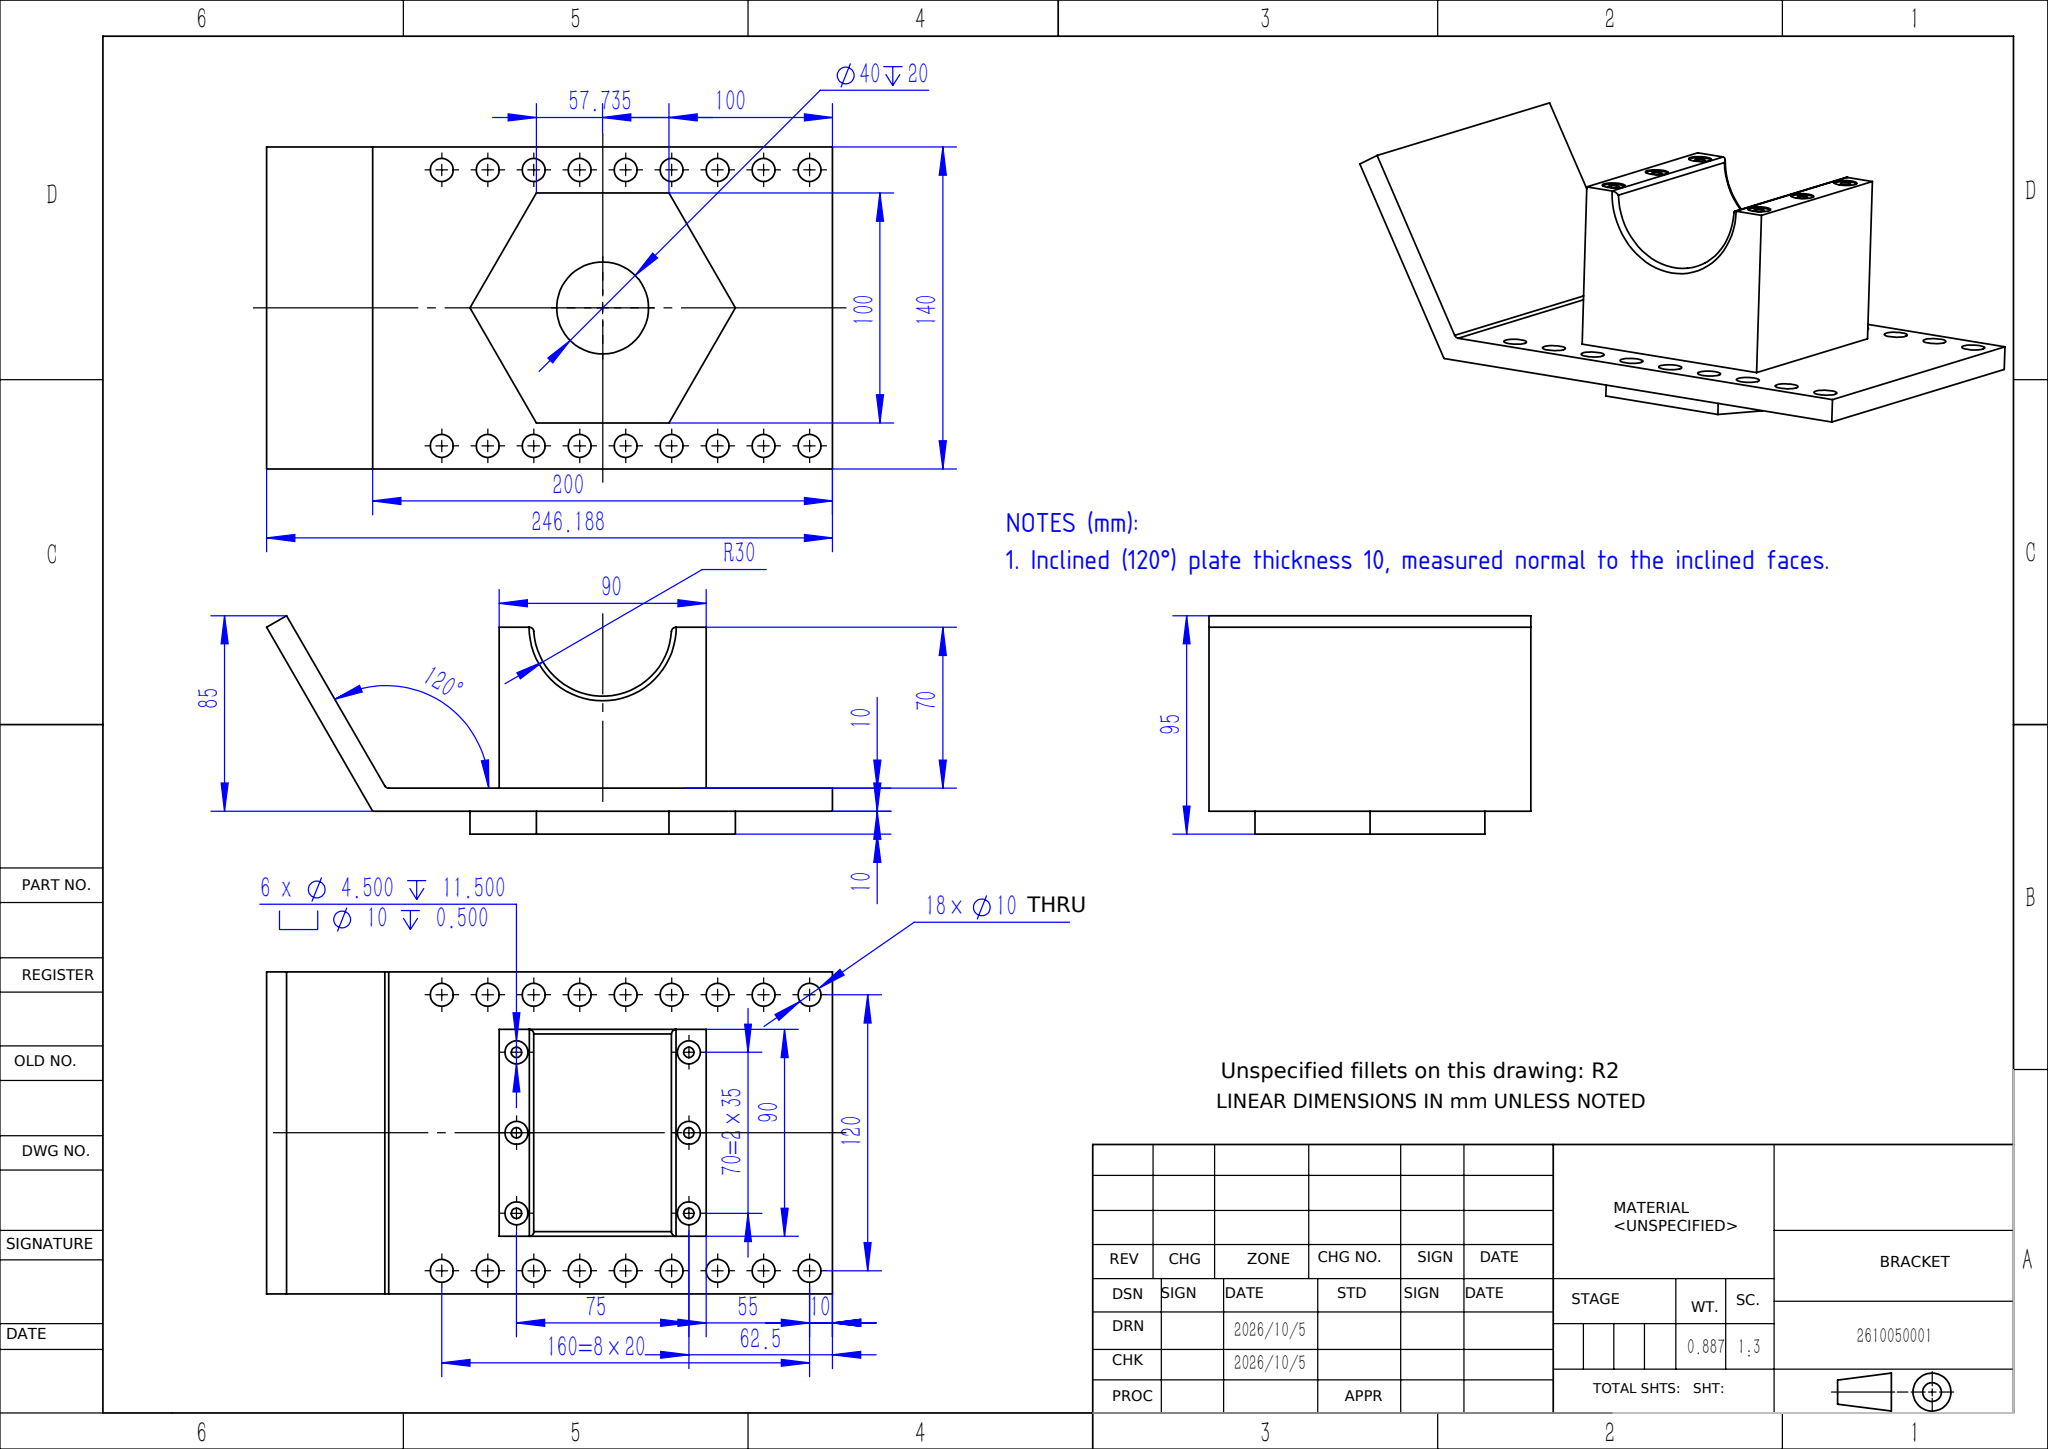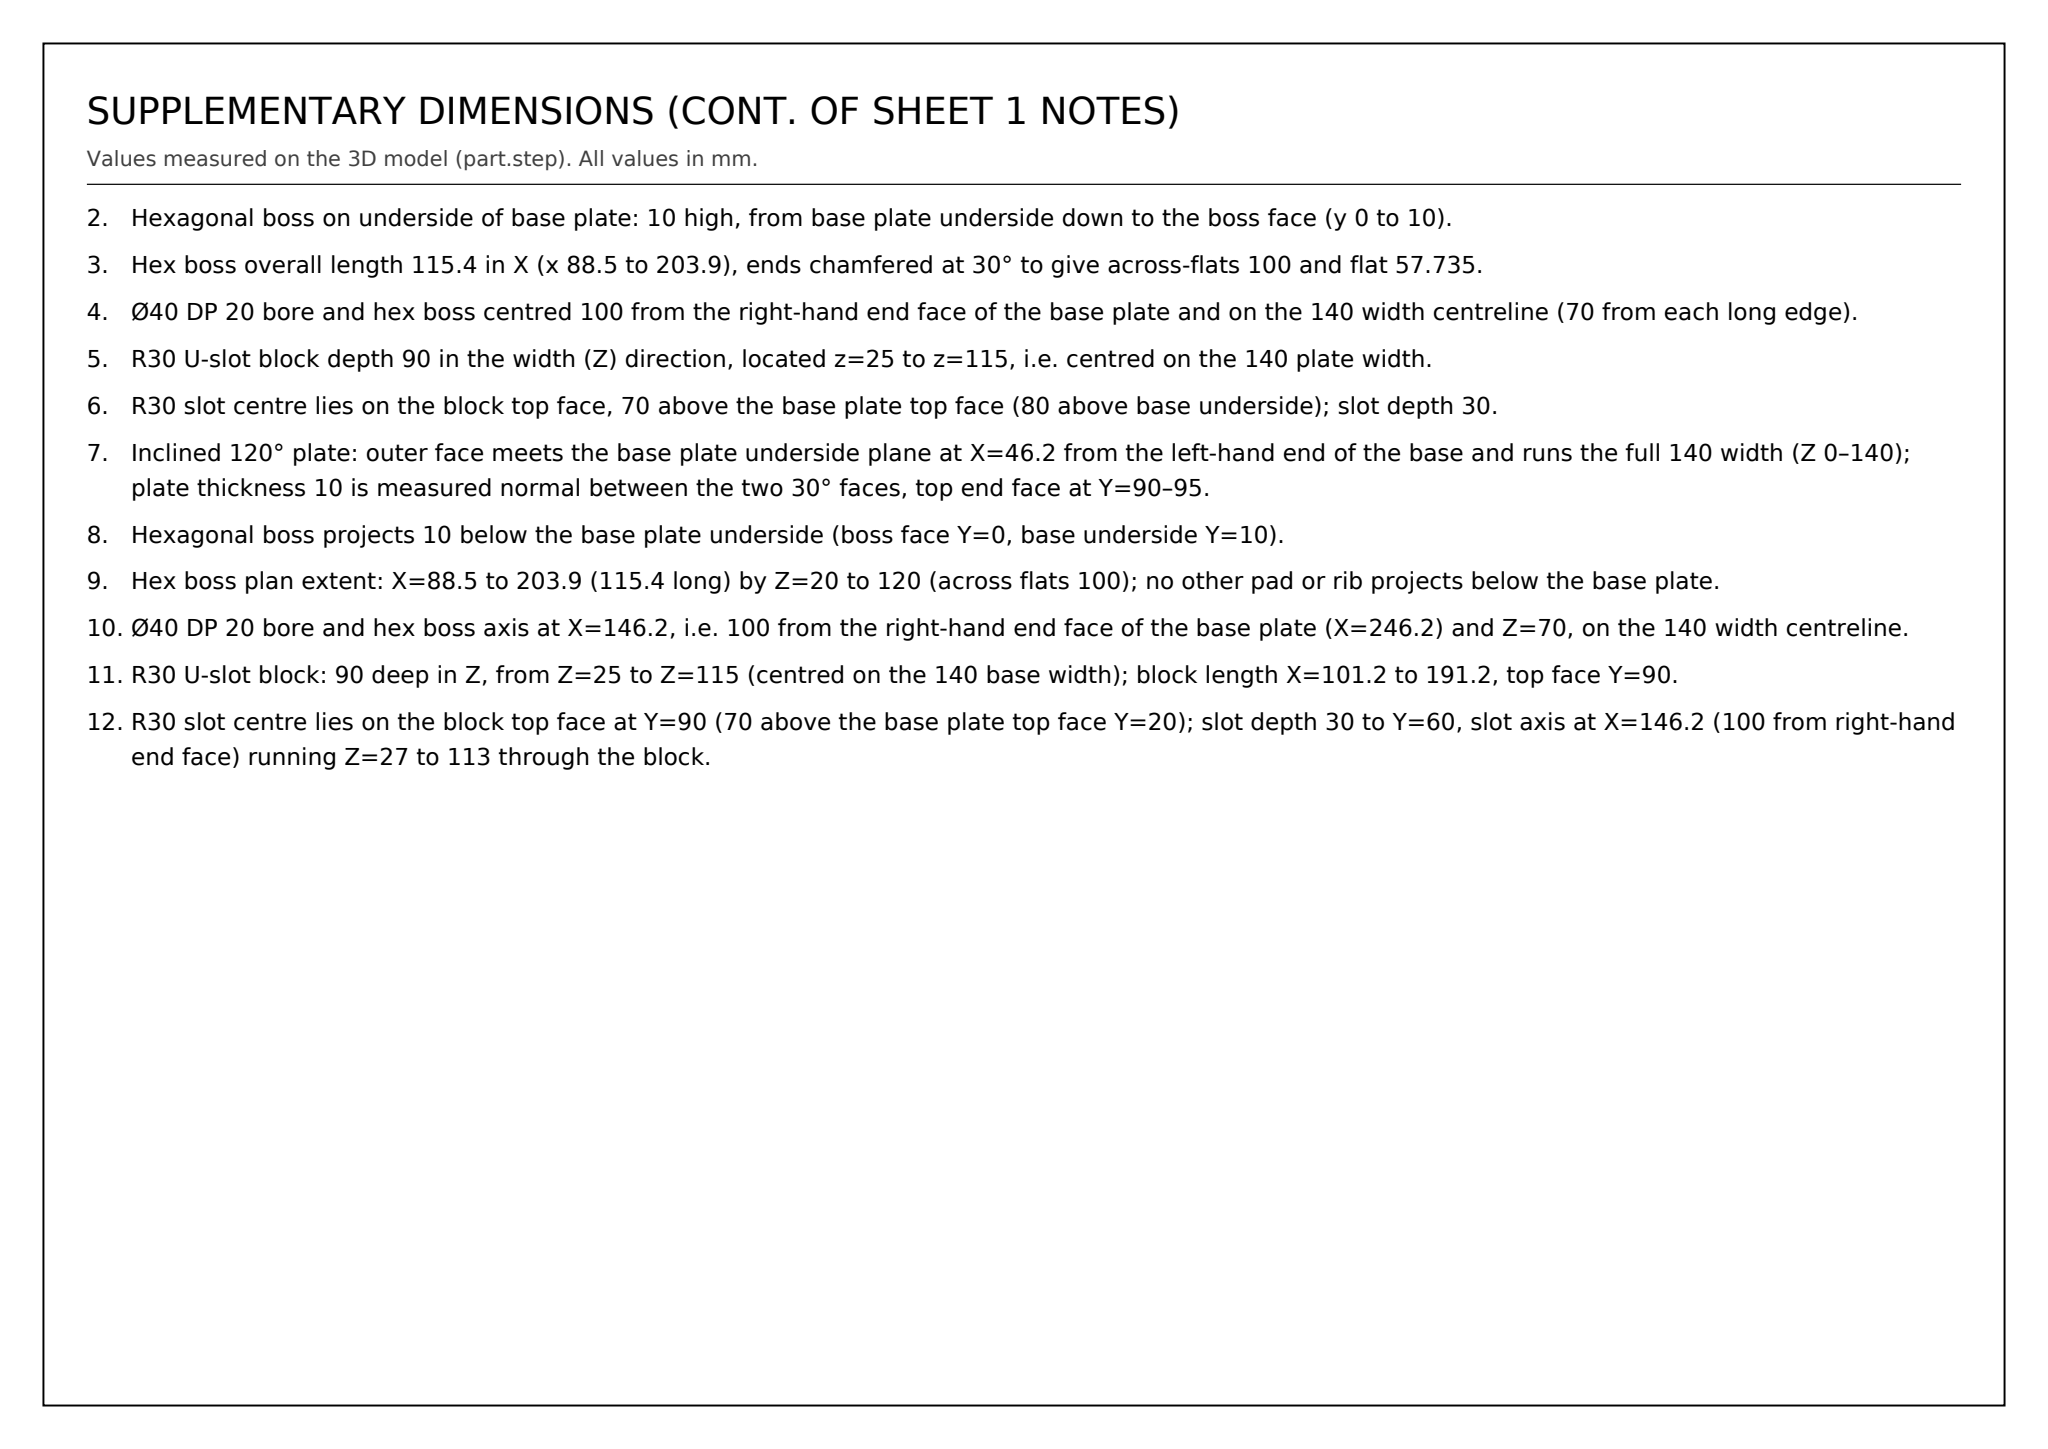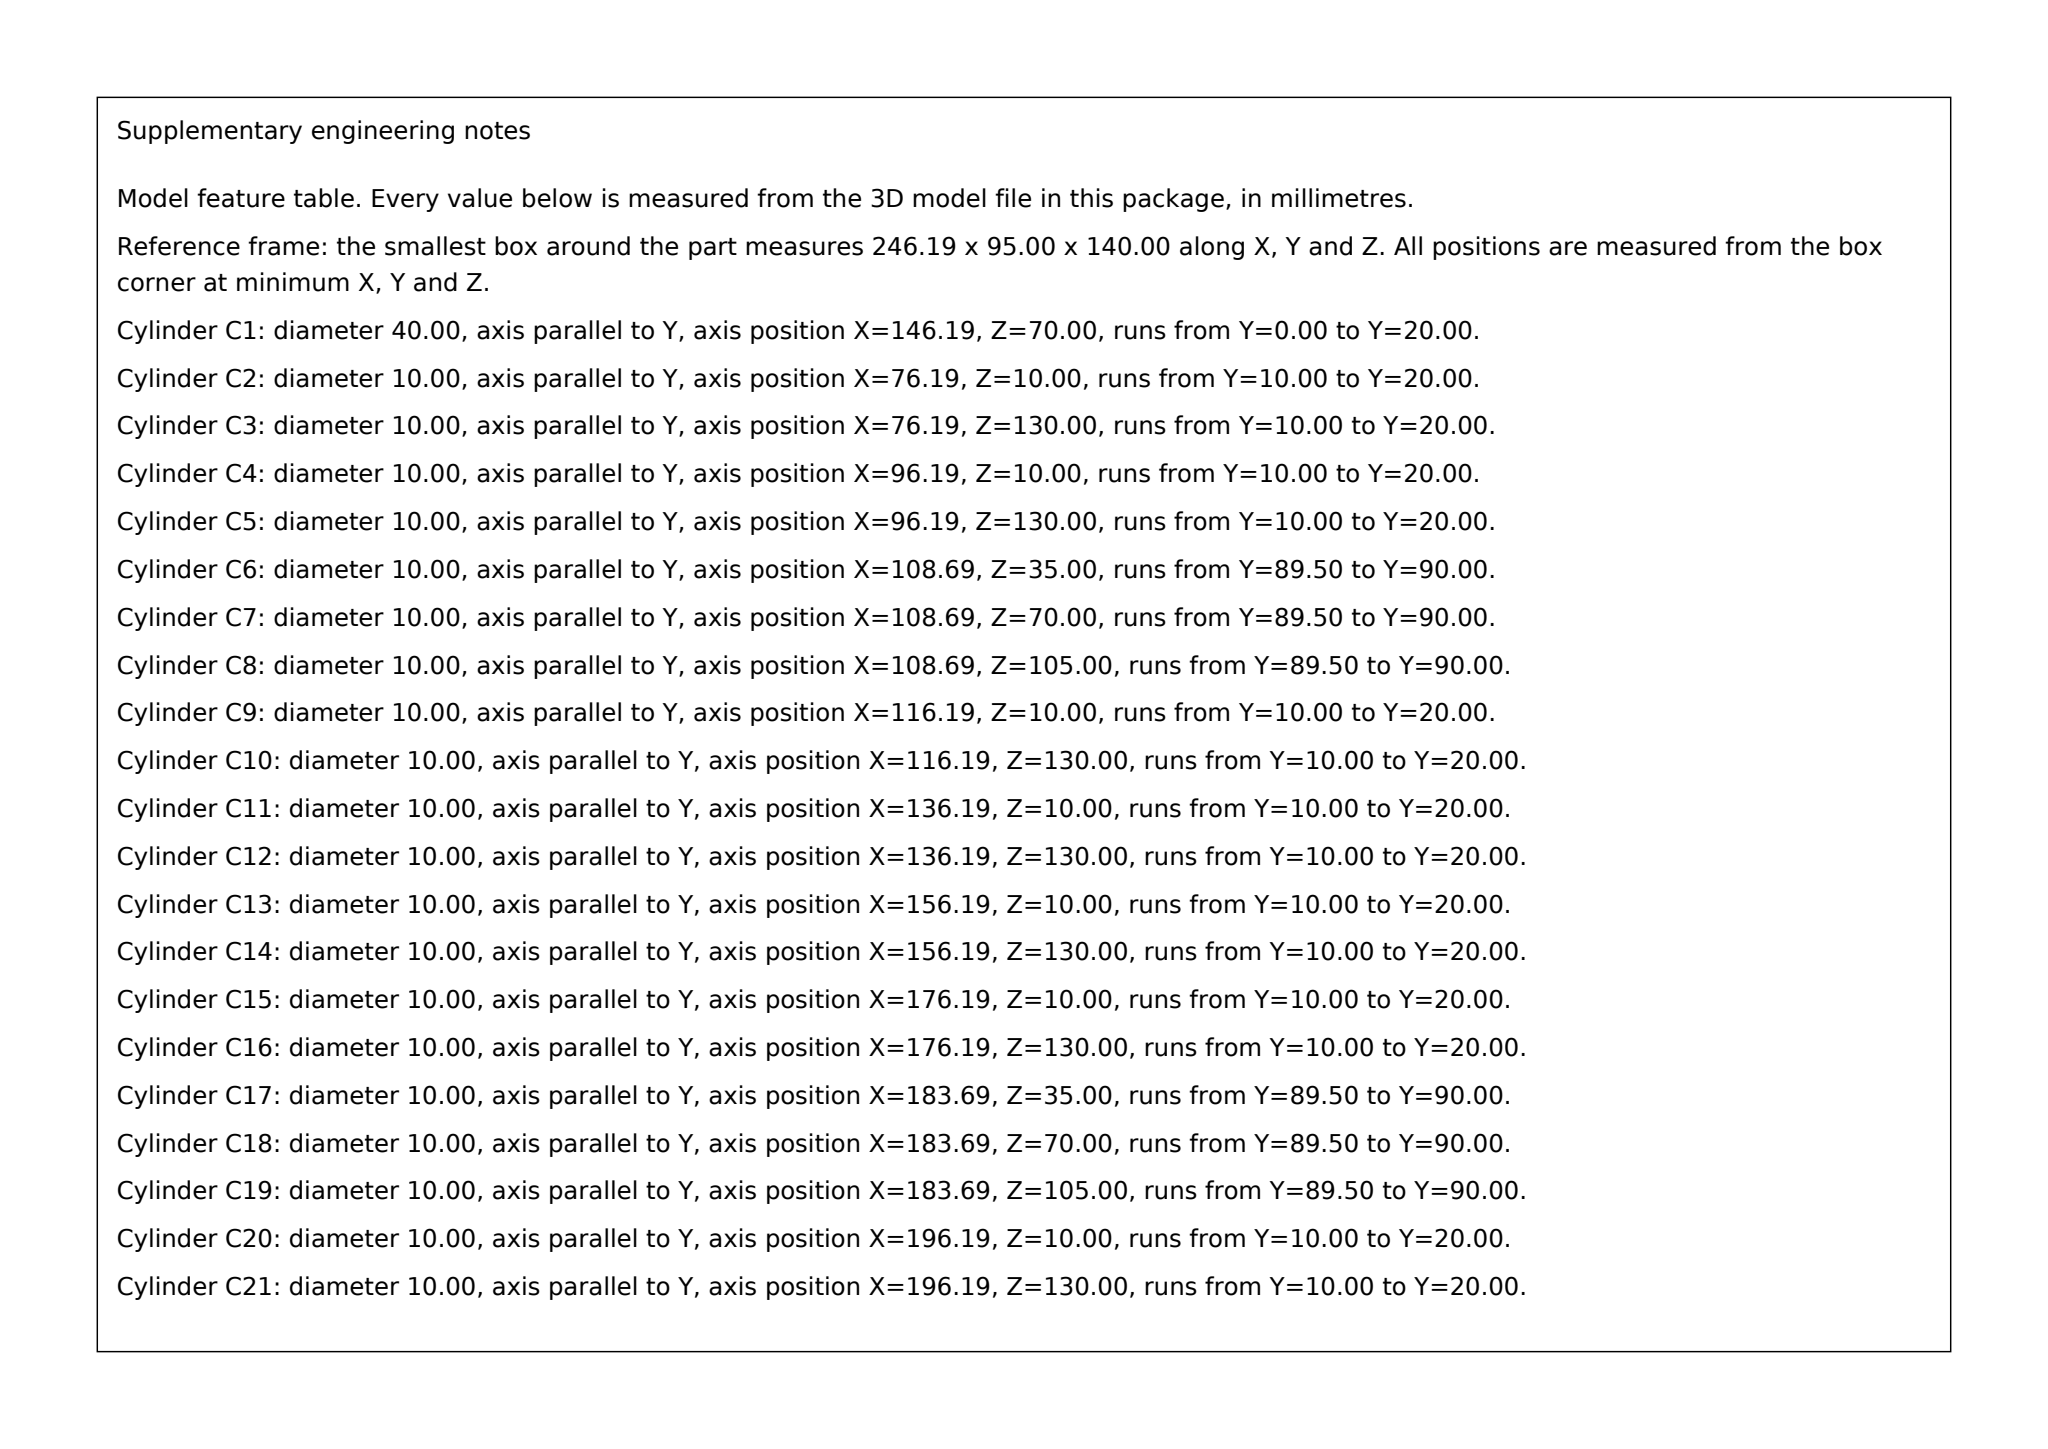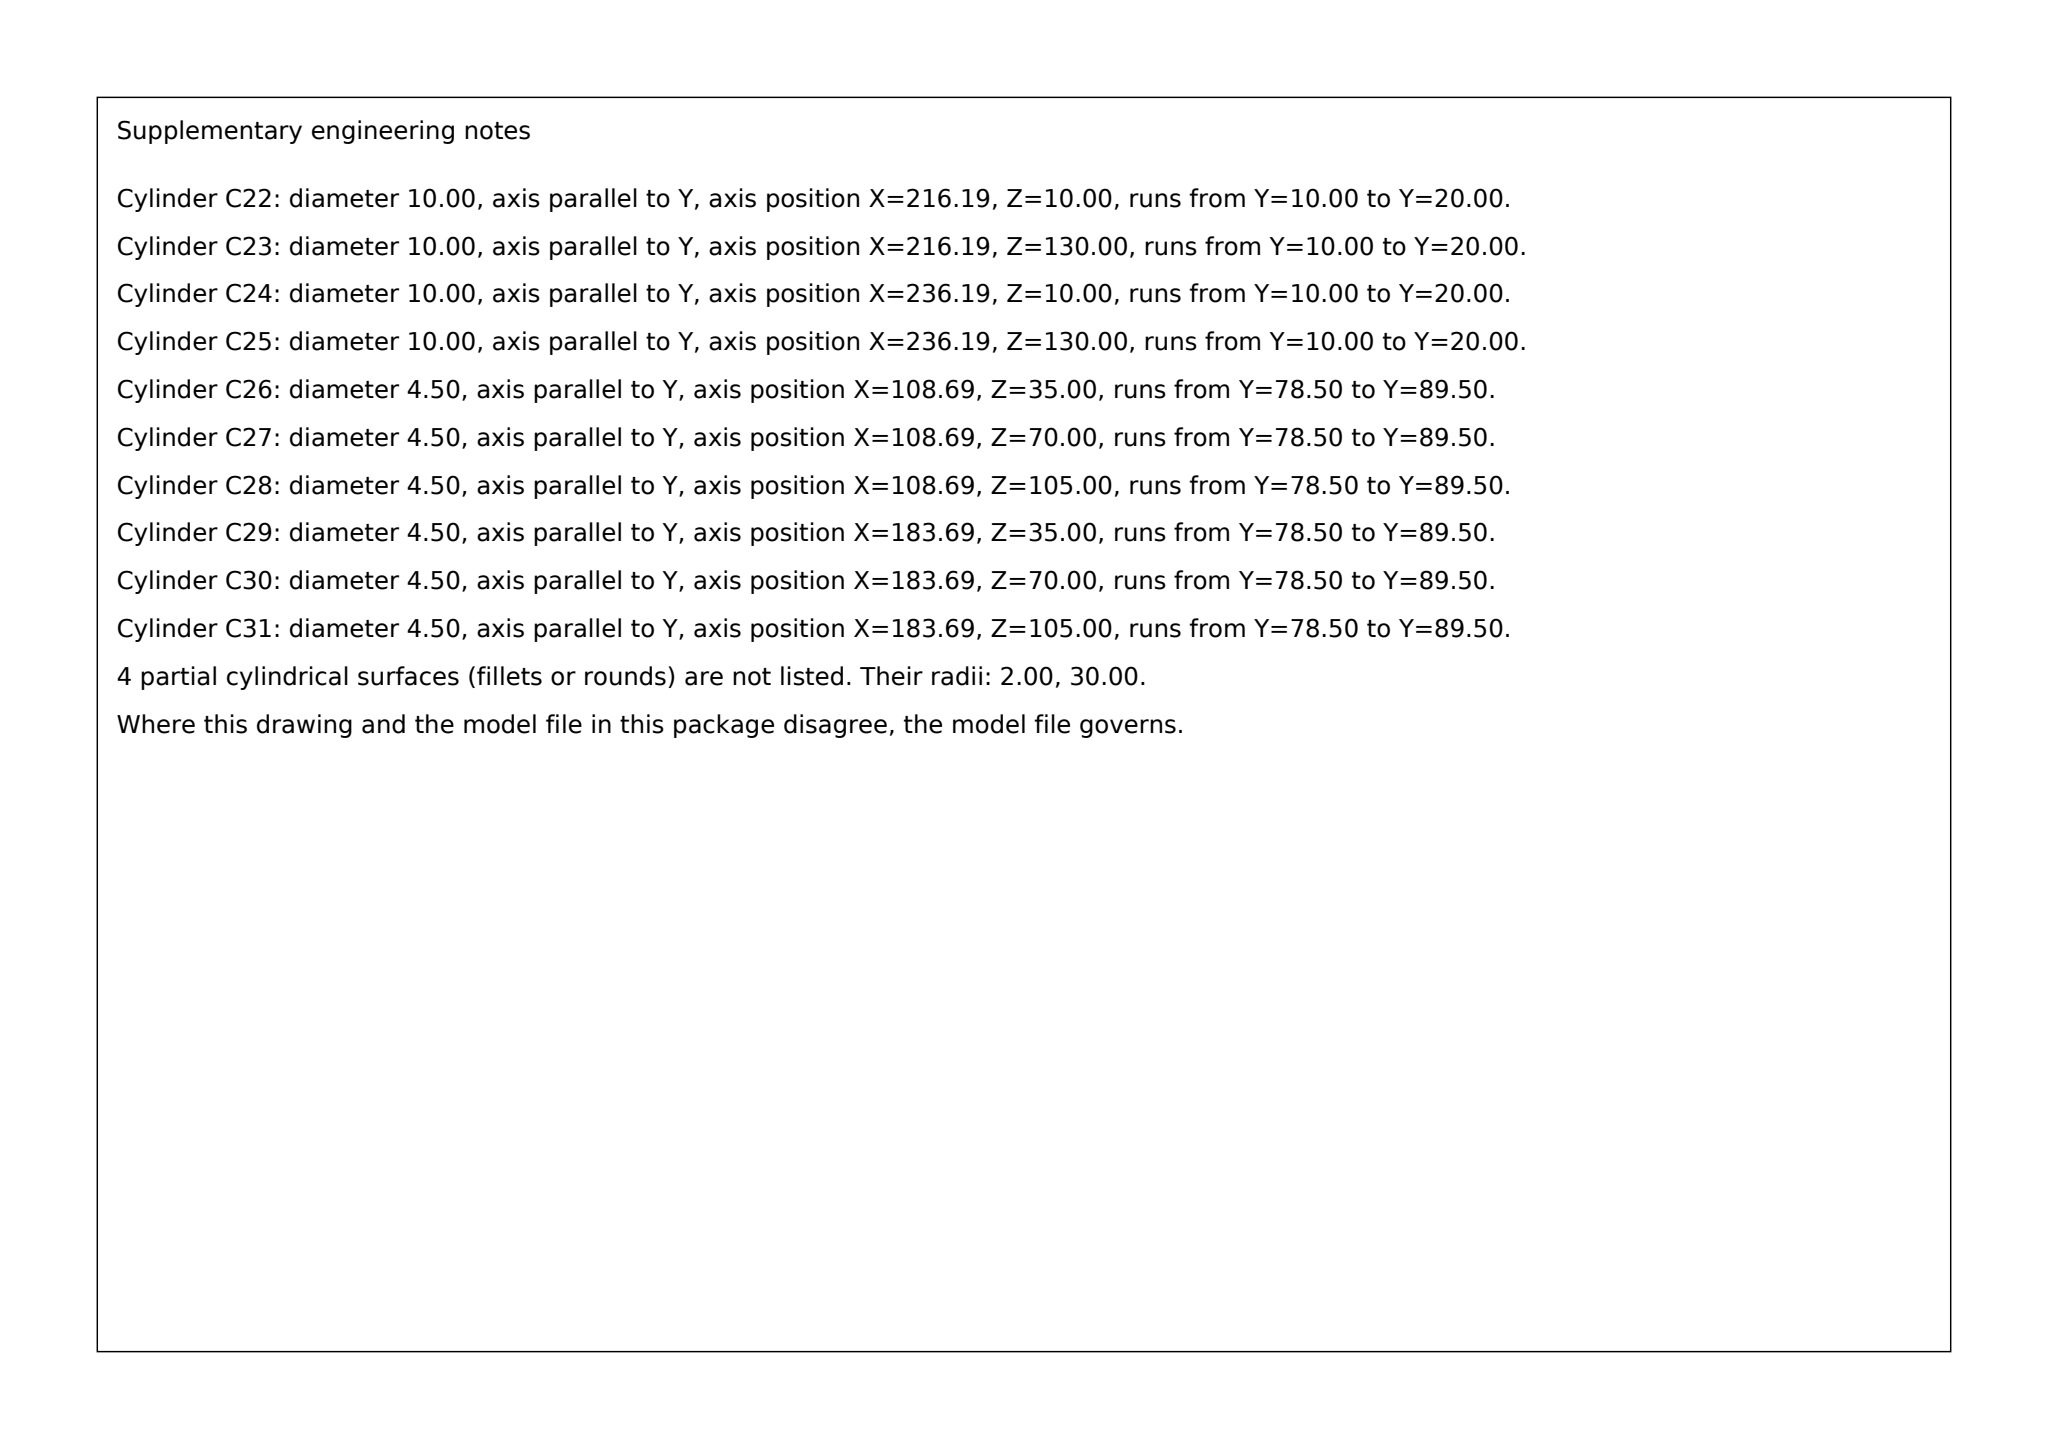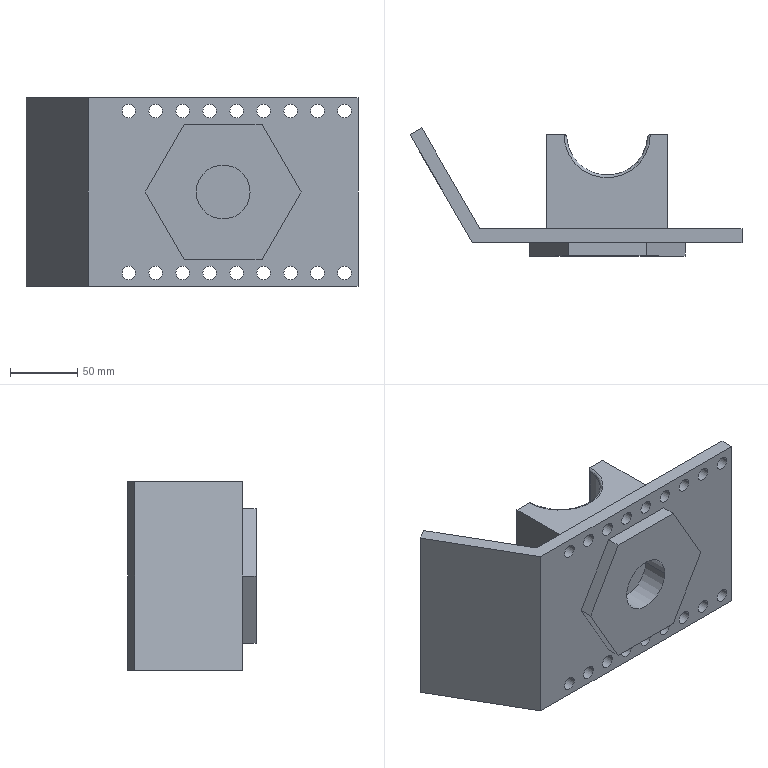Part | SolidWorks | mm | 1 solid | 108 faces | box 246.19 x 95 x 140 mm | volume 886742 mm3 | cylinder 66 | plane 28 | cone 12 | torus 2 | commonest cylinder face diameters 10 x48 4.5 x12 4 x3 40 x2 60 x1
Drawing notes:
Inclined (120°) plate thickness 10, measured normal to the inclined faces. | from the solid: Parallel inclined_planes at 30°/60°/90°: bbox_from [0,10,0] size [46.2,80,140] and bbox_from [8.7,21,0] size [42.7,74,140] — normal offset 10; end face inclined plane bbox_from [0,90,0] size [8.7,5,140].
Hexagonal boss on underside of base plate: 10 high, from base plate underside down to the boss face (y 0 to 10). | from the solid: axis_planes z-normal? -> y-normal planes: y=0 extent x[88.5,203.9] z[20,120] (boss face) and y=10 extent x[46.2,246.2] z[0,140] (base underside).
Hex boss overall length 115.4 in X (x 88.5 to 203.9), ends chamfered at 30° to give across-flats 100 and flat 57.735. | from the solid: inclined_planes [30,90,60] at bbox_from [88.5,0,20], [88.5,0,70], [175.1,0,20], [175.1,0,70], size [28.9,10,50]; plane y=0 extent x[88.5,203.9] z[20,120].
Ø40 DP 20 bore and hex boss centred 100 from the right-hand end face of the base plate and on the 140 width centreline (70 from each long edge). | from the solid: cylinder Ø40 axis y at [146.2, -, 70] from y=0 to 20; plane x=246.2 (right end face), plate z extent 0 to 140.
R30 U-slot block depth 90 in the width (Z) direction, located z=25 to z=115, i.e. centred on the 140 plate width. | from the solid: axis_planes z=25 and z=115, each extent x[101.2,191.2] y[20,90]; block side faces x=101.2 and x=191.2.
R30 slot centre lies on the block top face, 70 above the base plate top face (80 above base underside); slot depth 30. | from the solid: concave arc Ø60 axis z at [146.2, 90] arc 173°; block top faces y=90; base plate top face y=20 extent x[53.1,246.2].
Inclined 120° plate: outer face meets the base plate underside plane at X=46.2 from the left-hand end of the base and runs the full 140 width (Z 0–140); plate thickness 10 is measured normal between the two 30° faces, top end face at Y=90–95. | from the solid: inclined_planes 30° pair: bbox_from [0,10,0] size [46.2,80,140] and bbox_from [8.7,21,0] size [42.7,74,140] (normal offset = 10); inclined plane 60° bbox_from [0,90,0]
Hexagonal boss projects 10 below the base plate underside (boss face Y=0, base underside Y=10). | from the solid: axis_planes y=0 extent x[88.5,203.9] z[20,120]; axis_planes y=10 extent x[46.2,246.2] z[0,140]
Hex boss plan extent: X=88.5 to 203.9 (115.4 long) by Z=20 to 120 (across flats 100); no other pad or rib projects below the base plate. | from the solid: axis_planes y=0 extent x[88.5,203.9] z[20,120]; inclined_planes 30° chamfers at bbox_from [88.5,0,20],[88.5,0,70],[175.1,0,20],[175.1,0,70]
Ø40 DP 20 bore and hex boss axis at X=146.2, i.e. 100 from the right-hand end face of the base plate (X=246.2) and Z=70, on the 140 width centreline. | from the solid: hole/bore dia 40 axis y at [146.2,null,70] from y0 to y20; axis_planes x=246.2 extent y[10,20] z[0,140]
R30 U-slot block: 90 deep in Z, from Z=25 to Z=115 (centred on the 140 base width); block length X=101.2 to 191.2, top face Y=90. | from the solid: axis_planes z=25 and z=115 extent x[101.2,191.2] y[20,90]; axis_planes x=101.2 and x=191.2 extent y[20,90] z[25,115]
R30 slot centre lies on the block top face at Y=90 (70 above the base plate top face Y=20); slot depth 30 to Y=60, slot axis at X=146.2 (100 from right-hand end face) running Z=27 to 113 through the block. | from the solid: concave arc dia 60 axis z at [146.2,90] from z=27 to z=113, 173°; axis_planes y=20 extent x[53.1,246.2] z[0,140]
build123d program:
from build123d import *

# Parameters (mm, degrees)
EXTRUDE_THIN1_DEPTH                                 = 70
BOSS_EXTRUDE1_DEPTH                                 = 10
SKETCH3_R                                           = 20
CUT_EXTRUDE1_DEPTH                                  = 233.218
SKETCH4_R                                           = 5
CUT_EXTRUDE2_DEPTH                                  = 229.309
SKETCH5_W                                           = 90
SKETCH5_H                                           = 90
BOSS_EXTRUDE2_DEPTH                                 = 70
CUT_EXTRUDE3_DEPTH                                  = 246.866
CYLINDRICAL_COUNTERSUNK_HOLE_FOR_M4_HEX_D           = 4.5
CYLINDRICAL_COUNTERSUNK_HOLE_FOR_M4_HEX_DEPTH       = 11.5
CYLINDRICAL_COUNTERSUNK_HOLE_FOR_M4_HEX_CBORE_D     = 10
CYLINDRICAL_COUNTERSUNK_HOLE_FOR_M4_HEX_CBORE_DEPTH = 0.5
CYLINDRICAL_COUNTERSUNK_HOLE_FOR_M4_HEX_TIP         = 1.352
FILLET1_R                                           = 2


with BuildPart() as part:
    # Sketch1 → Extrude-Thin1 (new, symmetric)
    with BuildSketch(Plane.XY):
        Polygon((200, 0), (0, 0), (-46.188, 80), (-37.528, 85), (5.774, 10), (200, 10), align=None)
    extrude(amount=EXTRUDE_THIN1_DEPTH, both=True)

    # Sketch2 → Boss-Extrude1 (add)
    with BuildSketch(Plane.XZ):
        Polygon((128.868, 50), (71.132, 50), (42.265, 0), (71.132, -50), (128.868, -50), (157.735, 0), align=None)
    extrude(amount=BOSS_EXTRUDE1_DEPTH)

    # Sketch3 → Cut-Extrude1 (cut, through all)
    with BuildSketch(Plane.XZ.offset(10)):
        with Locations((100, 0)):
            Circle(SKETCH3_R)
    extrude(amount=-CUT_EXTRUDE1_DEPTH, mode=Mode.SUBTRACT)

    # Sketch4 → Cut-Extrude2 (cut, through all)
    with BuildSketch(Plane.XZ):
        with Locations((190, 60)):
            Circle(SKETCH4_R)
        with Locations((170, 60)):
            Circle(SKETCH4_R)
        with Locations((150, 60)):
            Circle(SKETCH4_R)
        with Locations((130, 60)):
            Circle(SKETCH4_R)
        with Locations((110, 60)):
            Circle(SKETCH4_R)
        with Locations((90, 60)):
            Circle(SKETCH4_R)
        with Locations((70, 60)):
            Circle(SKETCH4_R)
        with Locations((50, 60)):
            Circle(SKETCH4_R)
        with Locations((30, 60)):
            Circle(SKETCH4_R)
        with Locations((170, -60)):
            Circle(SKETCH4_R)
        with Locations((150, -60)):
            Circle(SKETCH4_R)
        with Locations((130, -60)):
            Circle(SKETCH4_R)
        with Locations((110, -60)):
            Circle(SKETCH4_R)
        with Locations((90, -60)):
            Circle(SKETCH4_R)
        with Locations((70, -60)):
            Circle(SKETCH4_R)
        with Locations((50, -60)):
            Circle(SKETCH4_R)
        with Locations((30, -60)):
            Circle(SKETCH4_R)
        with Locations((190, -60)):
            Circle(SKETCH4_R)
    extrude(amount=-CUT_EXTRUDE2_DEPTH, mode=Mode.SUBTRACT)

    # Sketch5 → Boss-Extrude2 (add)
    with BuildSketch(Plane(origin=(0, 10, 0), x_dir=(1, 0, 0), z_dir=(0, 1, 0))):
        with Locations((100, 0)):
            Rectangle(SKETCH5_W, SKETCH5_H)
    extrude(amount=BOSS_EXTRUDE2_DEPTH)

    # Sketch6 → Cut-Extrude3 (cut, through all)
    with BuildSketch(Plane.XY.offset(45)):
        with BuildLine():
            Line((70, 80), (130, 80))
            ThreePointArc((130, 80), (100, 50), (70, 80))
        make_face()
    extrude(amount=-CUT_EXTRUDE3_DEPTH, mode=Mode.SUBTRACT)

    # Cylindrical Countersunk Hole for M4 Hex
    with Locations(Plane(origin=(0, 80, 0), x_dir=(1, 0, 0), z_dir=(0, 1, 0))):
        with Locations((62.5, 35), (62.5, 0), (62.5, -35), (137.5, 35), (137.5, 0), (137.5, -35)):
            CounterBoreHole(CYLINDRICAL_COUNTERSUNK_HOLE_FOR_M4_HEX_D / 2, CYLINDRICAL_COUNTERSUNK_HOLE_FOR_M4_HEX_CBORE_D / 2, CYLINDRICAL_COUNTERSUNK_HOLE_FOR_M4_HEX_CBORE_DEPTH, depth=CYLINDRICAL_COUNTERSUNK_HOLE_FOR_M4_HEX_DEPTH)
            with Locations((0, 0, -(CYLINDRICAL_COUNTERSUNK_HOLE_FOR_M4_HEX_DEPTH + CYLINDRICAL_COUNTERSUNK_HOLE_FOR_M4_HEX_TIP / 2))):  # 118° drill point
                Cone(0, CYLINDRICAL_COUNTERSUNK_HOLE_FOR_M4_HEX_D / 2, CYLINDRICAL_COUNTERSUNK_HOLE_FOR_M4_HEX_TIP, mode=Mode.SUBTRACT)

    # Fillet1
    fillet1_edges = [part.edges().sort_by_distance(p)[0] for p in [
        (130, 80, 0),
        (70, 80, 0),
        (100, 50, -45),
        (100, 50, 45),
        (5.774, 10, 0),
    ]]
    fillet(fillet1_edges, radius=FILLET1_R)


solid = part.part